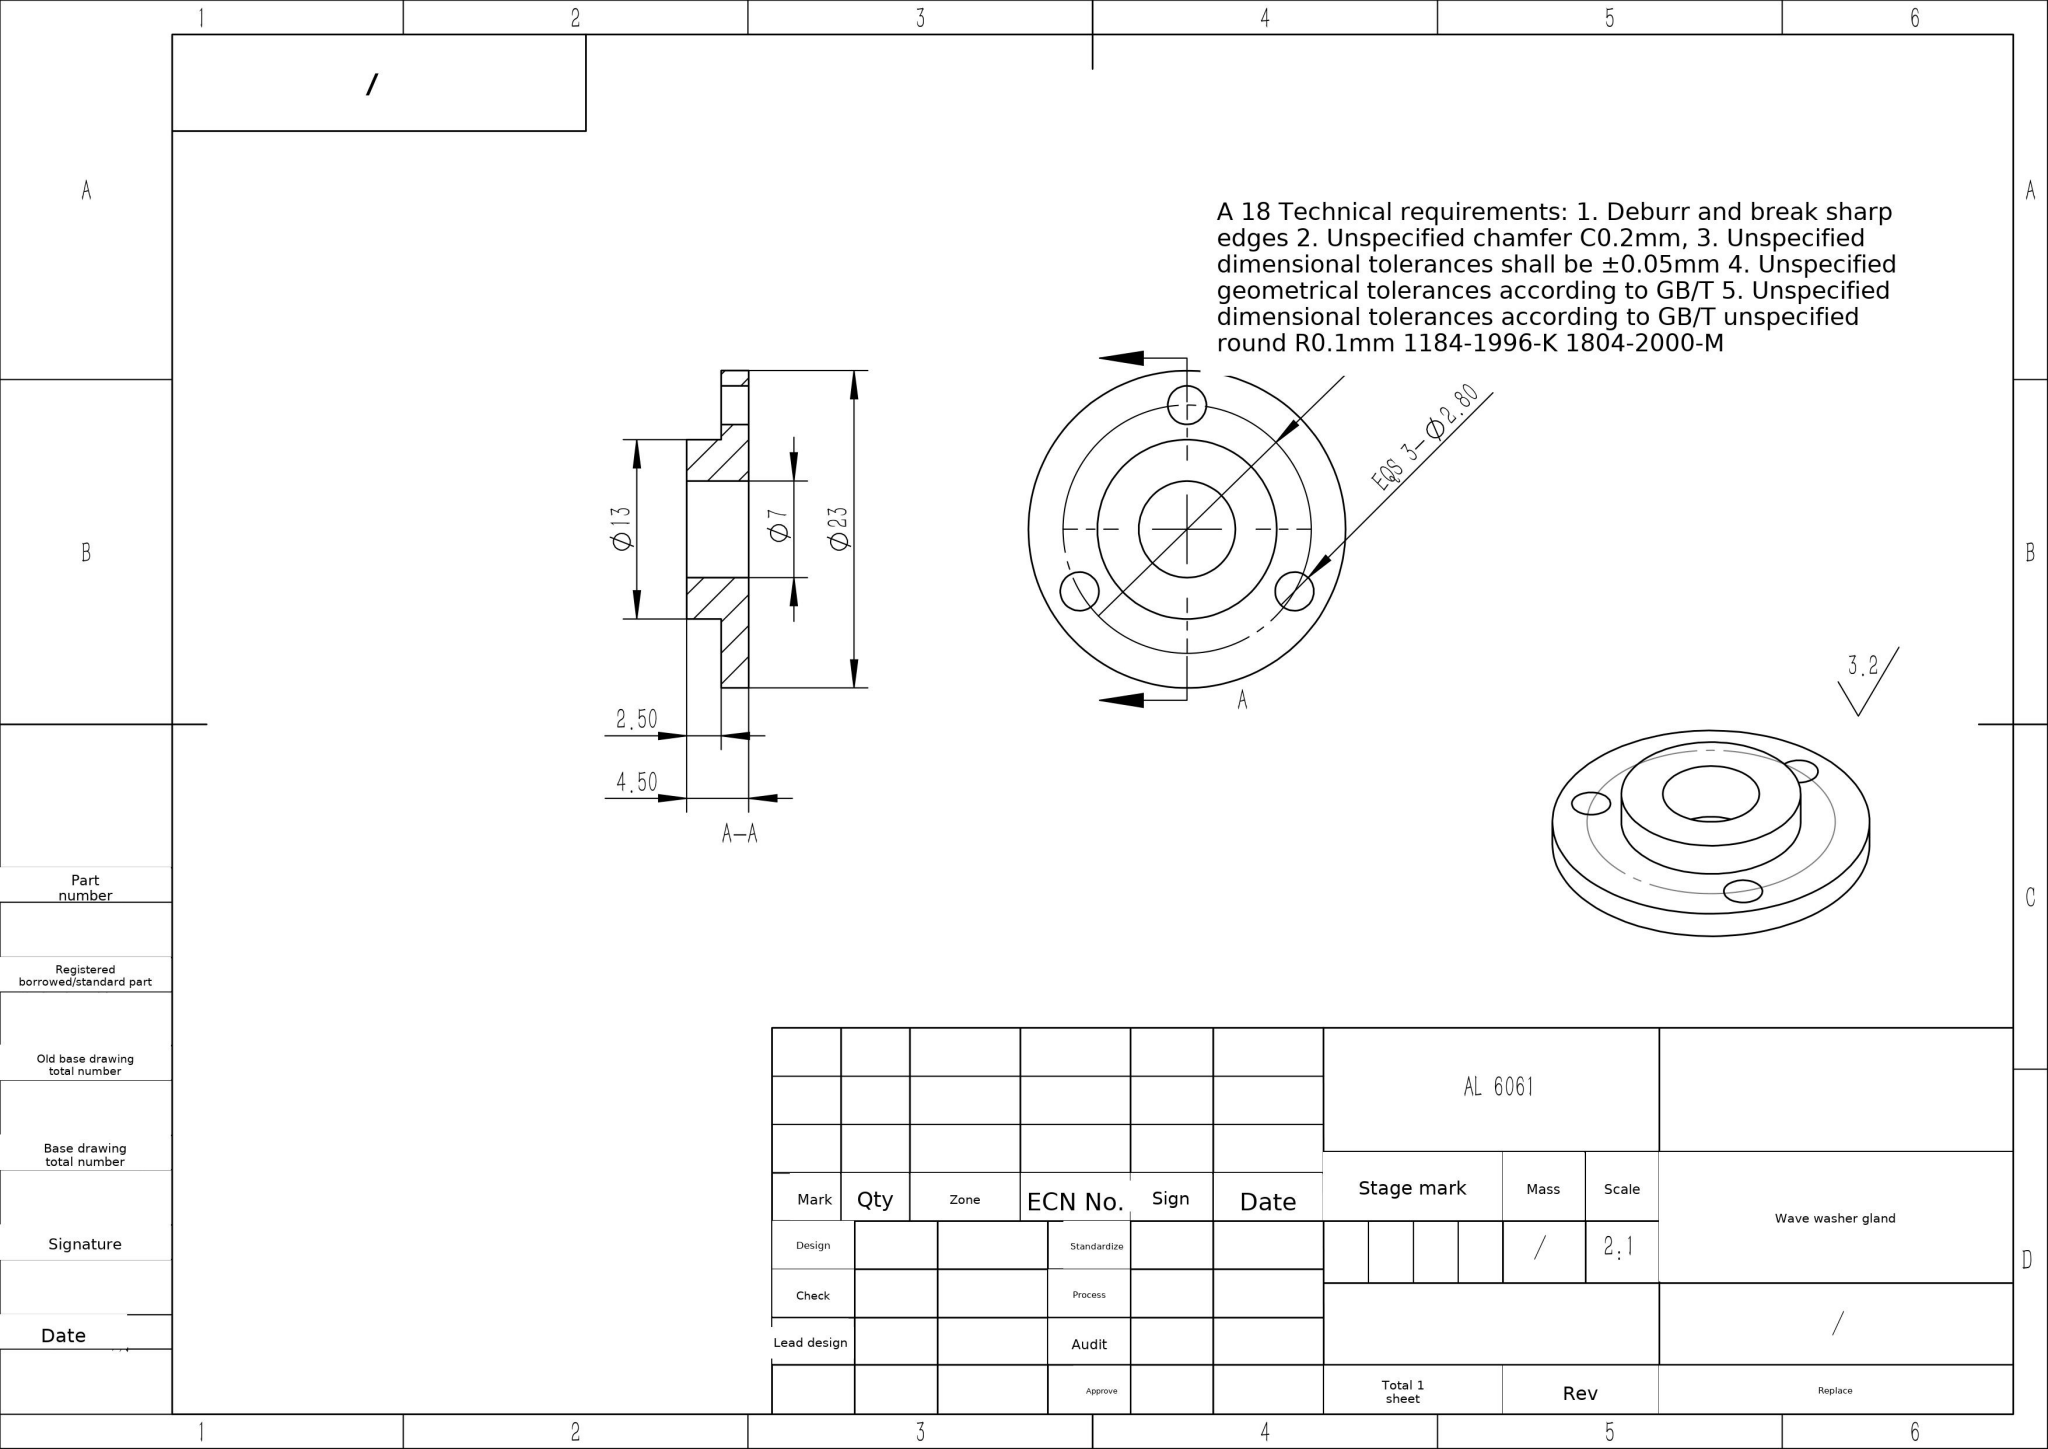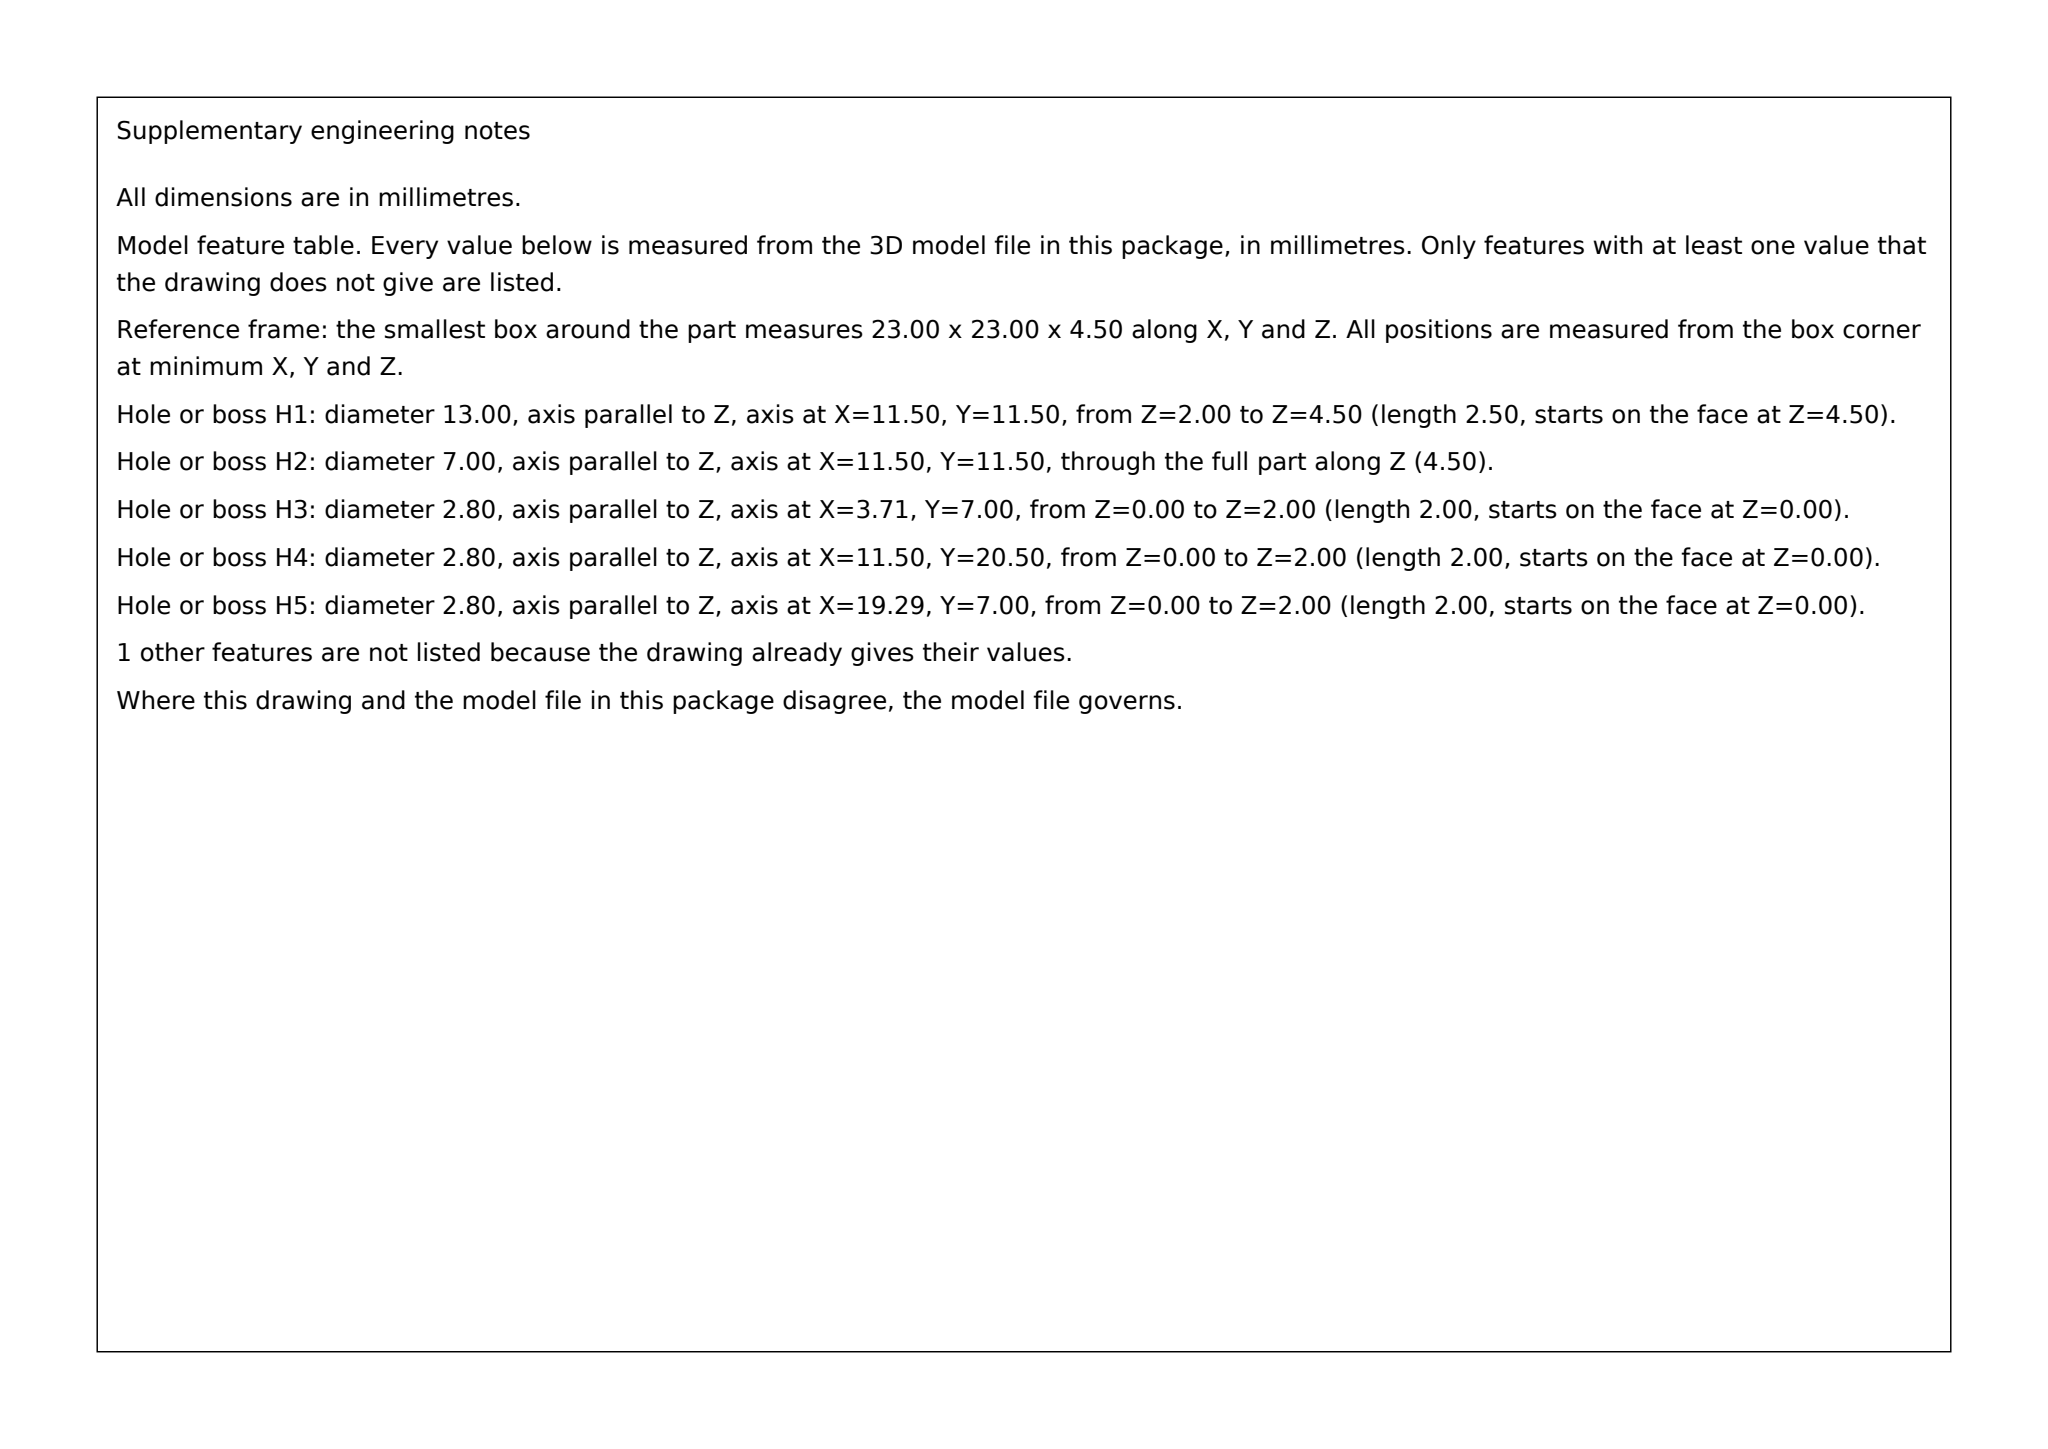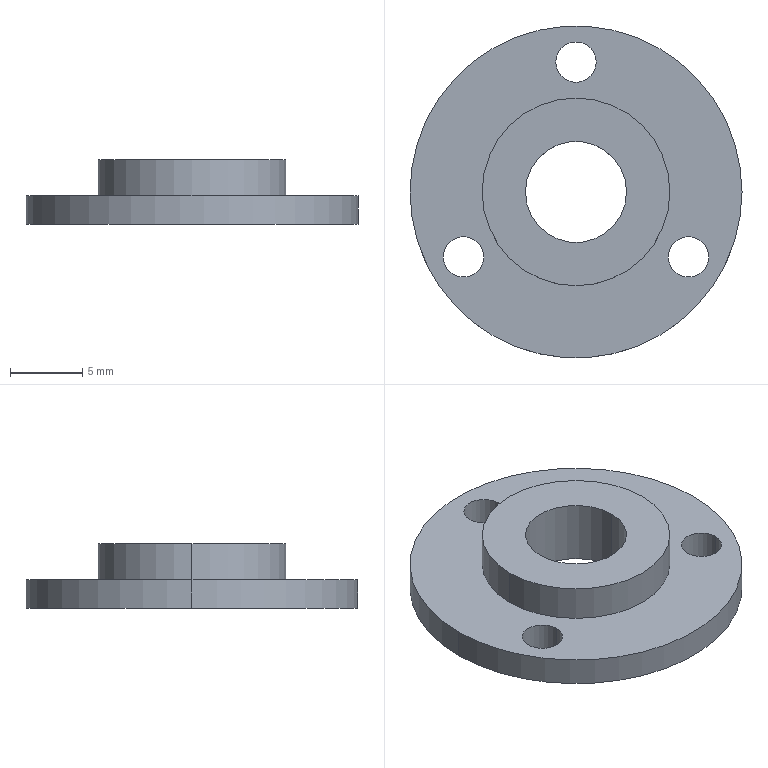Part | SolidWorks | mm | material AL 6061 | 1 solid | 15 faces | box 23 x 23 x 4.5 mm | volume 953 mm3 | cylinder 12 | plane 3 | commonest cylinder face diameters 2.8 x6 23 x2 7 x2 13 x2
build123d program:
from build123d import *
from build123d.topology import SkipClean

# Parameters (mm, degrees)
SKETCH1_R           = 6.5
SKETCH1_R_2         = 3.5
BOSS_EXTRUDE1_DEPTH = 2.5
BOSS_EXTRUDE2_START = 2
SKETCH2_R           = 11.5
SKETCH2_R_2         = 3.5
BOSS_EXTRUDE2_DEPTH = 2
SKETCH6_R           = 1.4
CUT_EXTRUDE1_DEPTH  = 17.454


with BuildPart() as part:
    # Sketch1 → Boss-Extrude1 (new body)
    with BuildSketch(Plane.XY):
        Circle(SKETCH1_R)
        Circle(SKETCH1_R_2, mode=Mode.SUBTRACT)
    extrude(amount=BOSS_EXTRUDE1_DEPTH)

    # Sketch2 → Boss-Extrude2 (add)
    with SkipClean():  # the faces are left unmerged after this step: merging them gives an invalid solid
        with BuildSketch(Plane(origin=(0, 0, 0), x_dir=(-1, 0, 0), z_dir=(0, 0, -1)).offset(BOSS_EXTRUDE2_START)):
            Circle(SKETCH2_R)
            Circle(SKETCH2_R_2, mode=Mode.SUBTRACT)
        extrude(amount=-BOSS_EXTRUDE2_DEPTH)

    # Sketch6 → Cut-Extrude1 (cut, through all)
    with SkipClean():  # the faces are left unmerged after this step: merging them gives an invalid solid
        with BuildSketch(Plane.XY):
            with Locations((0, 9)):
                Circle(SKETCH6_R)
            with Locations((7.794, -4.5)):
                Circle(SKETCH6_R)
            with Locations((-7.794, -4.5)):
                Circle(SKETCH6_R)
        extrude(amount=-CUT_EXTRUDE1_DEPTH, mode=Mode.SUBTRACT)


solid = part.part
STEP:
#1=CARTESIAN_POINT('',(-1.4,9.,-2.));
#2=VERTEX_POINT('',#1);
#3=CARTESIAN_POINT('',(1.4,9.,-2.));
#4=VERTEX_POINT('',#3);
#5=CARTESIAN_POINT('',(0.,9.,-2.));
#6=DIRECTION('',(0.,0.,1.));
#7=DIRECTION('',(1.,0.,0.));
#8=AXIS2_PLACEMENT_3D('',#5,#6,#7);
#9=CIRCLE('',#8,1.4);
#10=EDGE_CURVE('',#2,#4,#9,.T.);
#11=ORIENTED_EDGE('',*,*,#10,.F.);
#12=CARTESIAN_POINT('',(-1.4,9.,0.));
#13=VERTEX_POINT('',#12);
#14=CARTESIAN_POINT('',(-1.4,9.,-2.));
#15=DIRECTION('',(0.,0.,1.));
#16=VECTOR('',#15,1000.);
#17=LINE('',#14,#16);
#18=EDGE_CURVE('',#2,#13,#17,.T.);
#19=ORIENTED_EDGE('',*,*,#18,.T.);
#20=CARTESIAN_POINT('',(1.4,9.,0.));
#21=VERTEX_POINT('',#20);
#22=CARTESIAN_POINT('',(0.,9.,0.));
#23=DIRECTION('',(0.,0.,1.));
#24=DIRECTION('',(1.,0.,0.));
#25=AXIS2_PLACEMENT_3D('',#22,#23,#24);
#26=CIRCLE('',#25,1.4);
#27=EDGE_CURVE('',#13,#21,#26,.T.);
#28=ORIENTED_EDGE('',*,*,#27,.T.);
#29=CARTESIAN_POINT('',(1.4,9.,-2.));
#30=DIRECTION('',(0.,0.,1.));
#31=VECTOR('',#30,1000.);
#32=LINE('',#29,#31);
#33=EDGE_CURVE('',#4,#21,#32,.T.);
#34=ORIENTED_EDGE('',*,*,#33,.F.);
#35=EDGE_LOOP('',(#11,#19,#28,#34));
#36=FACE_OUTER_BOUND('',#35,.T.);
#37=CARTESIAN_POINT('',(0.,9.,-2.));
#38=DIRECTION('',(0.,0.,1.));
#39=DIRECTION('',(1.,0.,0.));
#40=AXIS2_PLACEMENT_3D('',#37,#38,#39);
#41=CYLINDRICAL_SURFACE('',#40,1.4);
#42=ADVANCED_FACE('',(#36),#41,.F.);
#43=CARTESIAN_POINT('',(6.394,-4.5,-2.));
#44=VERTEX_POINT('',#43);
#45=CARTESIAN_POINT('',(9.194,-4.5,-2.));
#46=VERTEX_POINT('',#45);
#47=CARTESIAN_POINT('',(7.794,-4.5,-2.));
#48=DIRECTION('',(0.,0.,1.));
#49=DIRECTION('',(1.,0.,0.));
#50=AXIS2_PLACEMENT_3D('',#47,#48,#49);
#51=CIRCLE('',#50,1.4);
#52=EDGE_CURVE('',#44,#46,#51,.T.);
#53=ORIENTED_EDGE('',*,*,#52,.F.);
#54=CARTESIAN_POINT('',(6.394,-4.5,0.));
#55=VERTEX_POINT('',#54);
#56=CARTESIAN_POINT('',(6.394,-4.5,-2.));
#57=DIRECTION('',(0.,0.,1.));
#58=VECTOR('',#57,1000.);
#59=LINE('',#56,#58);
#60=EDGE_CURVE('',#44,#55,#59,.T.);
#61=ORIENTED_EDGE('',*,*,#60,.T.);
#62=CARTESIAN_POINT('',(9.194,-4.5,0.));
#63=VERTEX_POINT('',#62);
#64=CARTESIAN_POINT('',(7.794,-4.5,0.));
#65=DIRECTION('',(0.,0.,1.));
#66=DIRECTION('',(1.,0.,0.));
#67=AXIS2_PLACEMENT_3D('',#64,#65,#66);
#68=CIRCLE('',#67,1.4);
#69=EDGE_CURVE('',#55,#63,#68,.T.);
#70=ORIENTED_EDGE('',*,*,#69,.T.);
#71=CARTESIAN_POINT('',(9.194,-4.5,-2.));
#72=DIRECTION('',(0.,0.,1.));
#73=VECTOR('',#72,1000.);
#74=LINE('',#71,#73);
#75=EDGE_CURVE('',#46,#63,#74,.T.);
#76=ORIENTED_EDGE('',*,*,#75,.F.);
#77=EDGE_LOOP('',(#53,#61,#70,#76));
#78=FACE_OUTER_BOUND('',#77,.T.);
#79=CARTESIAN_POINT('',(7.794,-4.5,-2.));
#80=DIRECTION('',(0.,0.,1.));
#81=DIRECTION('',(1.,0.,0.));
#82=AXIS2_PLACEMENT_3D('',#79,#80,#81);
#83=CYLINDRICAL_SURFACE('',#82,1.4);
#84=ADVANCED_FACE('',(#78),#83,.F.);
#85=CARTESIAN_POINT('',(-9.194,-4.5,-2.));
#86=VERTEX_POINT('',#85);
#87=CARTESIAN_POINT('',(-6.394,-4.5,-2.));
#88=VERTEX_POINT('',#87);
#89=CARTESIAN_POINT('',(-7.794,-4.5,-2.));
#90=DIRECTION('',(0.,0.,1.));
#91=DIRECTION('',(1.,0.,0.));
#92=AXIS2_PLACEMENT_3D('',#89,#90,#91);
#93=CIRCLE('',#92,1.4);
#94=EDGE_CURVE('',#86,#88,#93,.T.);
#95=ORIENTED_EDGE('',*,*,#94,.F.);
#96=CARTESIAN_POINT('',(-9.194,-4.5,0.));
#97=VERTEX_POINT('',#96);
#98=CARTESIAN_POINT('',(-9.194,-4.5,-2.));
#99=DIRECTION('',(0.,0.,1.));
#100=VECTOR('',#99,1000.);
#101=LINE('',#98,#100);
#102=EDGE_CURVE('',#86,#97,#101,.T.);
#103=ORIENTED_EDGE('',*,*,#102,.T.);
#104=CARTESIAN_POINT('',(-6.394,-4.5,0.));
#105=VERTEX_POINT('',#104);
#106=CARTESIAN_POINT('',(-7.794,-4.5,0.));
#107=DIRECTION('',(0.,0.,1.));
#108=DIRECTION('',(1.,0.,0.));
#109=AXIS2_PLACEMENT_3D('',#106,#107,#108);
#110=CIRCLE('',#109,1.4);
#111=EDGE_CURVE('',#97,#105,#110,.T.);
#112=ORIENTED_EDGE('',*,*,#111,.T.);
#113=CARTESIAN_POINT('',(-6.394,-4.5,-2.));
#114=DIRECTION('',(0.,0.,1.));
#115=VECTOR('',#114,1000.);
#116=LINE('',#113,#115);
#117=EDGE_CURVE('',#88,#105,#116,.T.);
#118=ORIENTED_EDGE('',*,*,#117,.F.);
#119=EDGE_LOOP('',(#95,#103,#112,#118));
#120=FACE_OUTER_BOUND('',#119,.T.);
#121=CARTESIAN_POINT('',(-7.794,-4.5,-2.));
#122=DIRECTION('',(0.,0.,1.));
#123=DIRECTION('',(1.,0.,0.));
#124=AXIS2_PLACEMENT_3D('',#121,#122,#123);
#125=CYLINDRICAL_SURFACE('',#124,1.4);
#126=ADVANCED_FACE('',(#120),#125,.F.);
#127=CARTESIAN_POINT('',(-11.5,0.,-2.));
#128=VERTEX_POINT('',#127);
#129=CARTESIAN_POINT('',(11.5,0.,-2.));
#130=VERTEX_POINT('',#129);
#131=CARTESIAN_POINT('',(0.,0.,-2.));
#132=DIRECTION('',(0.,0.,-1.));
#133=DIRECTION('',(-1.,0.,0.));
#134=AXIS2_PLACEMENT_3D('',#131,#132,#133);
#135=CIRCLE('',#134,11.5);
#136=EDGE_CURVE('',#128,#130,#135,.T.);
#137=ORIENTED_EDGE('',*,*,#136,.F.);
#138=CARTESIAN_POINT('',(-11.5,0.,0.));
#139=VERTEX_POINT('',#138);
#140=CARTESIAN_POINT('',(-11.5,0.,-2.));
#141=DIRECTION('',(0.,0.,1.));
#142=VECTOR('',#141,1000.);
#143=LINE('',#140,#142);
#144=EDGE_CURVE('',#128,#139,#143,.T.);
#145=ORIENTED_EDGE('',*,*,#144,.T.);
#146=CARTESIAN_POINT('',(11.5,0.,0.));
#147=VERTEX_POINT('',#146);
#148=CARTESIAN_POINT('',(0.,0.,0.));
#149=DIRECTION('',(0.,0.,-1.));
#150=DIRECTION('',(-1.,0.,0.));
#151=AXIS2_PLACEMENT_3D('',#148,#149,#150);
#152=CIRCLE('',#151,11.5);
#153=EDGE_CURVE('',#139,#147,#152,.T.);
#154=ORIENTED_EDGE('',*,*,#153,.T.);
#155=CARTESIAN_POINT('',(11.5,0.,-2.));
#156=DIRECTION('',(0.,0.,1.));
#157=VECTOR('',#156,1000.);
#158=LINE('',#155,#157);
#159=EDGE_CURVE('',#130,#147,#158,.T.);
#160=ORIENTED_EDGE('',*,*,#159,.F.);
#161=EDGE_LOOP('',(#137,#145,#154,#160));
#162=FACE_OUTER_BOUND('',#161,.T.);
#163=CARTESIAN_POINT('',(0.,0.,-2.));
#164=DIRECTION('',(0.,0.,1.));
#165=DIRECTION('',(1.,0.,0.));
#166=AXIS2_PLACEMENT_3D('',#163,#164,#165);
#167=CYLINDRICAL_SURFACE('',#166,11.5);
#168=ADVANCED_FACE('',(#162),#167,.T.);
#169=CARTESIAN_POINT('',(-3.5,0.,2.5));
#170=VERTEX_POINT('',#169);
#171=CARTESIAN_POINT('',(3.5,0.,2.5));
#172=VERTEX_POINT('',#171);
#173=CARTESIAN_POINT('',(0.,0.,2.5));
#174=DIRECTION('',(0.,0.,1.));
#175=DIRECTION('',(1.,0.,0.));
#176=AXIS2_PLACEMENT_3D('',#173,#174,#175);
#177=CIRCLE('',#176,3.5);
#178=EDGE_CURVE('',#170,#172,#177,.T.);
#179=ORIENTED_EDGE('',*,*,#178,.T.);
#180=CARTESIAN_POINT('',(3.5,0.,-2.));
#181=VERTEX_POINT('',#180);
#182=CARTESIAN_POINT('',(3.5,0.,2.5));
#183=DIRECTION('',(0.,0.,-1.));
#184=VECTOR('',#183,1000.);
#185=LINE('',#182,#184);
#186=EDGE_CURVE('',#172,#181,#185,.T.);
#187=ORIENTED_EDGE('',*,*,#186,.T.);
#188=CARTESIAN_POINT('',(-3.5,0.,-2.));
#189=VERTEX_POINT('',#188);
#190=CARTESIAN_POINT('',(0.,0.,-2.));
#191=DIRECTION('',(0.,0.,-1.));
#192=DIRECTION('',(-1.,0.,0.));
#193=AXIS2_PLACEMENT_3D('',#190,#191,#192);
#194=CIRCLE('',#193,3.5);
#195=EDGE_CURVE('',#181,#189,#194,.T.);
#196=ORIENTED_EDGE('',*,*,#195,.T.);
#197=CARTESIAN_POINT('',(-3.5,0.,2.5));
#198=DIRECTION('',(0.,0.,-1.));
#199=VECTOR('',#198,1000.);
#200=LINE('',#197,#199);
#201=EDGE_CURVE('',#170,#189,#200,.T.);
#202=ORIENTED_EDGE('',*,*,#201,.F.);
#203=EDGE_LOOP('',(#179,#187,#196,#202));
#204=FACE_OUTER_BOUND('',#203,.T.);
#205=CARTESIAN_POINT('',(0.,0.,2.5));
#206=DIRECTION('',(0.,0.,-1.));
#207=DIRECTION('',(-1.,0.,0.));
#208=AXIS2_PLACEMENT_3D('',#205,#206,#207);
#209=CYLINDRICAL_SURFACE('',#208,3.5);
#210=ADVANCED_FACE('',(#204),#209,.F.);
#211=CARTESIAN_POINT('',(6.5,0.,2.5));
#212=VERTEX_POINT('',#211);
#213=CARTESIAN_POINT('',(-6.5,0.,2.5));
#214=VERTEX_POINT('',#213);
#215=CARTESIAN_POINT('',(0.,0.,2.5));
#216=DIRECTION('',(0.,0.,1.));
#217=DIRECTION('',(1.,0.,0.));
#218=AXIS2_PLACEMENT_3D('',#215,#216,#217);
#219=CIRCLE('',#218,6.5);
#220=EDGE_CURVE('',#212,#214,#219,.T.);
#221=ORIENTED_EDGE('',*,*,#220,.F.);
#222=CARTESIAN_POINT('',(6.5,0.,0.));
#223=VERTEX_POINT('',#222);
#224=CARTESIAN_POINT('',(6.5,0.,2.5));
#225=DIRECTION('',(0.,0.,-1.));
#226=VECTOR('',#225,1000.);
#227=LINE('',#224,#226);
#228=EDGE_CURVE('',#212,#223,#227,.T.);
#229=ORIENTED_EDGE('',*,*,#228,.T.);
#230=CARTESIAN_POINT('',(-6.5,0.,0.));
#231=VERTEX_POINT('',#230);
#232=CARTESIAN_POINT('',(0.,0.,0.));
#233=DIRECTION('',(0.,0.,1.));
#234=DIRECTION('',(1.,0.,0.));
#235=AXIS2_PLACEMENT_3D('',#232,#233,#234);
#236=CIRCLE('',#235,6.5);
#237=EDGE_CURVE('',#223,#231,#236,.T.);
#238=ORIENTED_EDGE('',*,*,#237,.T.);
#239=CARTESIAN_POINT('',(-6.5,0.,2.5));
#240=DIRECTION('',(0.,0.,-1.));
#241=VECTOR('',#240,1000.);
#242=LINE('',#239,#241);
#243=EDGE_CURVE('',#214,#231,#242,.T.);
#244=ORIENTED_EDGE('',*,*,#243,.F.);
#245=EDGE_LOOP('',(#221,#229,#238,#244));
#246=FACE_OUTER_BOUND('',#245,.T.);
#247=CARTESIAN_POINT('',(0.,0.,2.5));
#248=DIRECTION('',(0.,0.,-1.));
#249=DIRECTION('',(-1.,0.,0.));
#250=AXIS2_PLACEMENT_3D('',#247,#248,#249);
#251=CYLINDRICAL_SURFACE('',#250,6.5);
#252=ADVANCED_FACE('',(#246),#251,.T.);
#253=CARTESIAN_POINT('',(0.,0.,2.5));
#254=DIRECTION('',(0.,0.,1.));
#255=DIRECTION('',(1.,0.,0.));
#256=AXIS2_PLACEMENT_3D('',#253,#254,#255);
#257=CIRCLE('',#256,6.5);
#258=EDGE_CURVE('',#214,#212,#257,.T.);
#259=ORIENTED_EDGE('',*,*,#258,.T.);
#260=ORIENTED_EDGE('',*,*,#220,.T.);
#261=EDGE_LOOP('',(#259,#260));
#262=FACE_OUTER_BOUND('',#261,.T.);
#263=ORIENTED_EDGE('',*,*,#178,.F.);
#264=CARTESIAN_POINT('',(0.,0.,2.5));
#265=DIRECTION('',(0.,0.,1.));
#266=DIRECTION('',(1.,0.,0.));
#267=AXIS2_PLACEMENT_3D('',#264,#265,#266);
#268=CIRCLE('',#267,3.5);
#269=EDGE_CURVE('',#172,#170,#268,.T.);
#270=ORIENTED_EDGE('',*,*,#269,.F.);
#271=EDGE_LOOP('',(#263,#270));
#272=FACE_BOUND('',#271,.T.);
#273=CARTESIAN_POINT('',(0.,0.,2.5));
#274=DIRECTION('',(0.,0.,1.));
#275=DIRECTION('',(1.,0.,0.));
#276=AXIS2_PLACEMENT_3D('',#273,#274,#275);
#277=PLANE('',#276);
#278=ADVANCED_FACE('',(#262,#272),#277,.T.);
#279=ORIENTED_EDGE('',*,*,#228,.F.);
#280=ORIENTED_EDGE('',*,*,#258,.F.);
#281=ORIENTED_EDGE('',*,*,#243,.T.);
#282=CARTESIAN_POINT('',(0.,0.,0.));
#283=DIRECTION('',(0.,0.,1.));
#284=DIRECTION('',(1.,0.,0.));
#285=AXIS2_PLACEMENT_3D('',#282,#283,#284);
#286=CIRCLE('',#285,6.5);
#287=EDGE_CURVE('',#231,#223,#286,.T.);
#288=ORIENTED_EDGE('',*,*,#287,.T.);
#289=EDGE_LOOP('',(#279,#280,#281,#288));
#290=FACE_OUTER_BOUND('',#289,.T.);
#291=CARTESIAN_POINT('',(0.,0.,2.5));
#292=DIRECTION('',(0.,0.,-1.));
#293=DIRECTION('',(-1.,0.,0.));
#294=AXIS2_PLACEMENT_3D('',#291,#292,#293);
#295=CYLINDRICAL_SURFACE('',#294,6.5);
#296=ADVANCED_FACE('',(#290),#295,.T.);
#297=ORIENTED_EDGE('',*,*,#186,.F.);
#298=ORIENTED_EDGE('',*,*,#269,.T.);
#299=ORIENTED_EDGE('',*,*,#201,.T.);
#300=CARTESIAN_POINT('',(0.,0.,-2.));
#301=DIRECTION('',(0.,0.,-1.));
#302=DIRECTION('',(-1.,0.,0.));
#303=AXIS2_PLACEMENT_3D('',#300,#301,#302);
#304=CIRCLE('',#303,3.5);
#305=EDGE_CURVE('',#189,#181,#304,.T.);
#306=ORIENTED_EDGE('',*,*,#305,.T.);
#307=EDGE_LOOP('',(#297,#298,#299,#306));
#308=FACE_OUTER_BOUND('',#307,.T.);
#309=CARTESIAN_POINT('',(0.,0.,2.5));
#310=DIRECTION('',(0.,0.,-1.));
#311=DIRECTION('',(-1.,0.,0.));
#312=AXIS2_PLACEMENT_3D('',#309,#310,#311);
#313=CYLINDRICAL_SURFACE('',#312,3.5);
#314=ADVANCED_FACE('',(#308),#313,.F.);
#315=CARTESIAN_POINT('',(0.,9.,-2.));
#316=DIRECTION('',(0.,0.,1.));
#317=DIRECTION('',(1.,0.,0.));
#318=AXIS2_PLACEMENT_3D('',#315,#316,#317);
#319=CIRCLE('',#318,1.4);
#320=EDGE_CURVE('',#4,#2,#319,.T.);
#321=ORIENTED_EDGE('',*,*,#320,.T.);
#322=ORIENTED_EDGE('',*,*,#10,.T.);
#323=EDGE_LOOP('',(#321,#322));
#324=FACE_BOUND('',#323,.T.);
#325=CARTESIAN_POINT('',(7.794,-4.5,-2.));
#326=DIRECTION('',(0.,0.,1.));
#327=DIRECTION('',(1.,0.,0.));
#328=AXIS2_PLACEMENT_3D('',#325,#326,#327);
#329=CIRCLE('',#328,1.4);
#330=EDGE_CURVE('',#46,#44,#329,.T.);
#331=ORIENTED_EDGE('',*,*,#330,.T.);
#332=ORIENTED_EDGE('',*,*,#52,.T.);
#333=EDGE_LOOP('',(#331,#332));
#334=FACE_BOUND('',#333,.T.);
#335=CARTESIAN_POINT('',(-7.794,-4.5,-2.));
#336=DIRECTION('',(0.,0.,1.));
#337=DIRECTION('',(1.,0.,0.));
#338=AXIS2_PLACEMENT_3D('',#335,#336,#337);
#339=CIRCLE('',#338,1.4);
#340=EDGE_CURVE('',#88,#86,#339,.T.);
#341=ORIENTED_EDGE('',*,*,#340,.T.);
#342=ORIENTED_EDGE('',*,*,#94,.T.);
#343=EDGE_LOOP('',(#341,#342));
#344=FACE_BOUND('',#343,.T.);
#345=CARTESIAN_POINT('',(0.,0.,-2.));
#346=DIRECTION('',(0.,0.,-1.));
#347=DIRECTION('',(-1.,0.,0.));
#348=AXIS2_PLACEMENT_3D('',#345,#346,#347);
#349=CIRCLE('',#348,11.5);
#350=EDGE_CURVE('',#130,#128,#349,.T.);
#351=ORIENTED_EDGE('',*,*,#350,.T.);
#352=ORIENTED_EDGE('',*,*,#136,.T.);
#353=EDGE_LOOP('',(#351,#352));
#354=FACE_OUTER_BOUND('',#353,.T.);
#355=ORIENTED_EDGE('',*,*,#305,.F.);
#356=ORIENTED_EDGE('',*,*,#195,.F.);
#357=EDGE_LOOP('',(#355,#356));
#358=FACE_BOUND('',#357,.T.);
#359=CARTESIAN_POINT('',(0.,0.,-2.));
#360=DIRECTION('',(0.,0.,-1.));
#361=DIRECTION('',(-1.,0.,0.));
#362=AXIS2_PLACEMENT_3D('',#359,#360,#361);
#363=PLANE('',#362);
#364=ADVANCED_FACE('',(#324,#334,#344,#354,#358),#363,.T.);
#365=CARTESIAN_POINT('',(0.,9.,0.));
#366=DIRECTION('',(0.,0.,1.));
#367=DIRECTION('',(1.,0.,0.));
#368=AXIS2_PLACEMENT_3D('',#365,#366,#367);
#369=CIRCLE('',#368,1.4);
#370=EDGE_CURVE('',#21,#13,#369,.T.);
#371=ORIENTED_EDGE('',*,*,#370,.F.);
#372=ORIENTED_EDGE('',*,*,#27,.F.);
#373=EDGE_LOOP('',(#371,#372));
#374=FACE_BOUND('',#373,.T.);
#375=CARTESIAN_POINT('',(7.794,-4.5,0.));
#376=DIRECTION('',(0.,0.,1.));
#377=DIRECTION('',(1.,0.,0.));
#378=AXIS2_PLACEMENT_3D('',#375,#376,#377);
#379=CIRCLE('',#378,1.4);
#380=EDGE_CURVE('',#63,#55,#379,.T.);
#381=ORIENTED_EDGE('',*,*,#380,.F.);
#382=ORIENTED_EDGE('',*,*,#69,.F.);
#383=EDGE_LOOP('',(#381,#382));
#384=FACE_BOUND('',#383,.T.);
#385=CARTESIAN_POINT('',(-7.794,-4.5,0.));
#386=DIRECTION('',(0.,0.,1.));
#387=DIRECTION('',(1.,0.,0.));
#388=AXIS2_PLACEMENT_3D('',#385,#386,#387);
#389=CIRCLE('',#388,1.4);
#390=EDGE_CURVE('',#105,#97,#389,.T.);
#391=ORIENTED_EDGE('',*,*,#390,.F.);
#392=ORIENTED_EDGE('',*,*,#111,.F.);
#393=EDGE_LOOP('',(#391,#392));
#394=FACE_BOUND('',#393,.T.);
#395=ORIENTED_EDGE('',*,*,#287,.F.);
#396=ORIENTED_EDGE('',*,*,#237,.F.);
#397=EDGE_LOOP('',(#395,#396));
#398=FACE_BOUND('',#397,.T.);
#399=CARTESIAN_POINT('',(0.,0.,0.));
#400=DIRECTION('',(0.,0.,-1.));
#401=DIRECTION('',(-1.,0.,0.));
#402=AXIS2_PLACEMENT_3D('',#399,#400,#401);
#403=CIRCLE('',#402,11.5);
#404=EDGE_CURVE('',#147,#139,#403,.T.);
#405=ORIENTED_EDGE('',*,*,#404,.F.);
#406=ORIENTED_EDGE('',*,*,#153,.F.);
#407=EDGE_LOOP('',(#405,#406));
#408=FACE_OUTER_BOUND('',#407,.T.);
#409=CARTESIAN_POINT('',(0.,0.,0.));
#410=DIRECTION('',(0.,0.,-1.));
#411=DIRECTION('',(-1.,0.,0.));
#412=AXIS2_PLACEMENT_3D('',#409,#410,#411);
#413=PLANE('',#412);
#414=ADVANCED_FACE('',(#374,#384,#394,#398,#408),#413,.F.);
#415=ORIENTED_EDGE('',*,*,#144,.F.);
#416=ORIENTED_EDGE('',*,*,#350,.F.);
#417=ORIENTED_EDGE('',*,*,#159,.T.);
#418=ORIENTED_EDGE('',*,*,#404,.T.);
#419=EDGE_LOOP('',(#415,#416,#417,#418));
#420=FACE_OUTER_BOUND('',#419,.T.);
#421=CARTESIAN_POINT('',(0.,0.,-2.));
#422=DIRECTION('',(0.,0.,1.));
#423=DIRECTION('',(1.,0.,0.));
#424=AXIS2_PLACEMENT_3D('',#421,#422,#423);
#425=CYLINDRICAL_SURFACE('',#424,11.5);
#426=ADVANCED_FACE('',(#420),#425,.T.);
#427=ORIENTED_EDGE('',*,*,#102,.F.);
#428=ORIENTED_EDGE('',*,*,#340,.F.);
#429=ORIENTED_EDGE('',*,*,#117,.T.);
#430=ORIENTED_EDGE('',*,*,#390,.T.);
#431=EDGE_LOOP('',(#427,#428,#429,#430));
#432=FACE_OUTER_BOUND('',#431,.T.);
#433=CARTESIAN_POINT('',(-7.794,-4.5,-2.));
#434=DIRECTION('',(0.,0.,1.));
#435=DIRECTION('',(1.,0.,0.));
#436=AXIS2_PLACEMENT_3D('',#433,#434,#435);
#437=CYLINDRICAL_SURFACE('',#436,1.4);
#438=ADVANCED_FACE('',(#432),#437,.F.);
#439=ORIENTED_EDGE('',*,*,#60,.F.);
#440=ORIENTED_EDGE('',*,*,#330,.F.);
#441=ORIENTED_EDGE('',*,*,#75,.T.);
#442=ORIENTED_EDGE('',*,*,#380,.T.);
#443=EDGE_LOOP('',(#439,#440,#441,#442));
#444=FACE_OUTER_BOUND('',#443,.T.);
#445=CARTESIAN_POINT('',(7.794,-4.5,-2.));
#446=DIRECTION('',(0.,0.,1.));
#447=DIRECTION('',(1.,0.,0.));
#448=AXIS2_PLACEMENT_3D('',#445,#446,#447);
#449=CYLINDRICAL_SURFACE('',#448,1.4);
#450=ADVANCED_FACE('',(#444),#449,.F.);
#451=ORIENTED_EDGE('',*,*,#18,.F.);
#452=ORIENTED_EDGE('',*,*,#320,.F.);
#453=ORIENTED_EDGE('',*,*,#33,.T.);
#454=ORIENTED_EDGE('',*,*,#370,.T.);
#455=EDGE_LOOP('',(#451,#452,#453,#454));
#456=FACE_OUTER_BOUND('',#455,.T.);
#457=CARTESIAN_POINT('',(0.,9.,-2.));
#458=DIRECTION('',(0.,0.,1.));
#459=DIRECTION('',(1.,0.,0.));
#460=AXIS2_PLACEMENT_3D('',#457,#458,#459);
#461=CYLINDRICAL_SURFACE('',#460,1.4);
#462=ADVANCED_FACE('',(#456),#461,.F.);
#463=CLOSED_SHELL('',(#42,#84,#126,#168,#210,#252,#278,#296,#314,#364,#414,#426,#438,#450,#462));
#464=MANIFOLD_SOLID_BREP('',#463);
#465=CARTESIAN_POINT('',(0.,0.,0.));
#466=DIRECTION('',(0.,0.,1.));
#467=DIRECTION('',(1.,0.,0.));
#468=AXIS2_PLACEMENT_3D('',#465,#466,#467);
#469=(LENGTH_UNIT()NAMED_UNIT(*)SI_UNIT(.MILLI.,.METRE.));
#470=UNCERTAINTY_MEASURE_WITH_UNIT(LENGTH_MEASURE(0.00001),#469,'','');
#471=(NAMED_UNIT(*)PLANE_ANGLE_UNIT()SI_UNIT($,.RADIAN.));
#472=(NAMED_UNIT(*)SI_UNIT($,.STERADIAN.)SOLID_ANGLE_UNIT());
#473=(GEOMETRIC_REPRESENTATION_CONTEXT(3)GLOBAL_UNCERTAINTY_ASSIGNED_CONTEXT((#470))GLOBAL_UNIT_ASSIGNED_CONTEXT((#469,#471,#472))REPRESENTATION_CONTEXT('',''));
#474=ADVANCED_BREP_SHAPE_REPRESENTATION('',(#464,#468),#473);